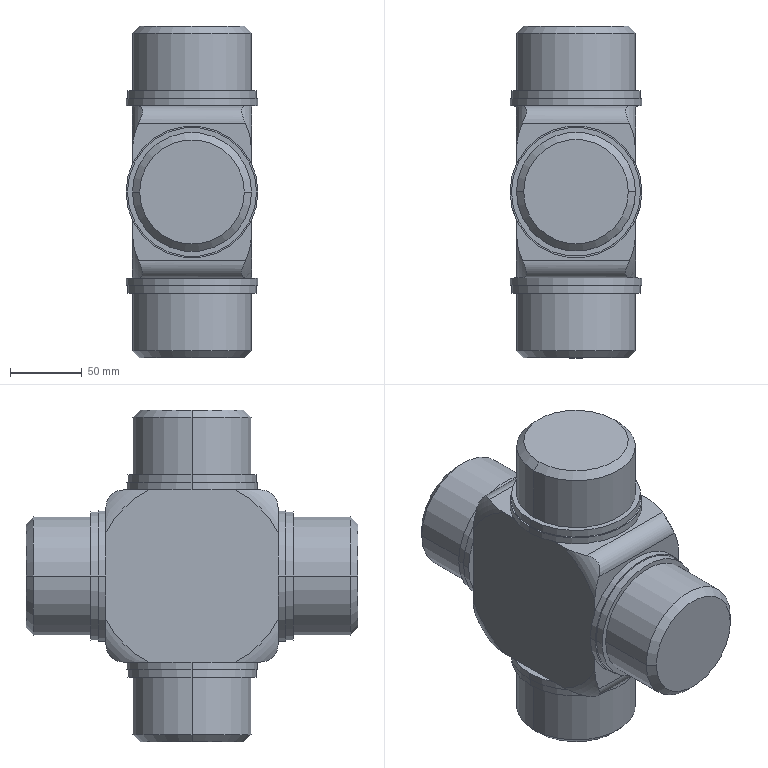Component | NX | CRUZ_587_PREDETERMINADO_COMO_MECANIZADA | 13 solids | 74 faces | volume 2420008 mm3 | plane 30 | cylinder 28 | torus 8 | cone 8 | commonest cylinder face diameters 90 x8 92 x8 83 x8 24 x4